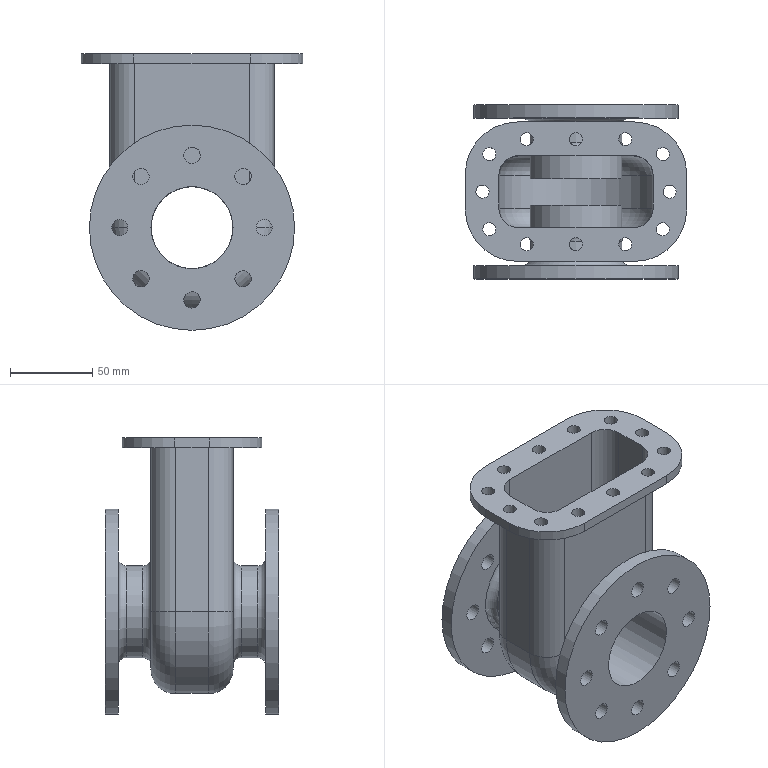Component | NX | VALVE_BODY | 1 solid | 78 faces | volume 334449 mm3 | cylinder 50 | plane 20 | torus 8 | commonest cylinder face diameters 10 x16 8 x12 64 x4 30 x4 56 x4 24 x4 125 x2 50 x2